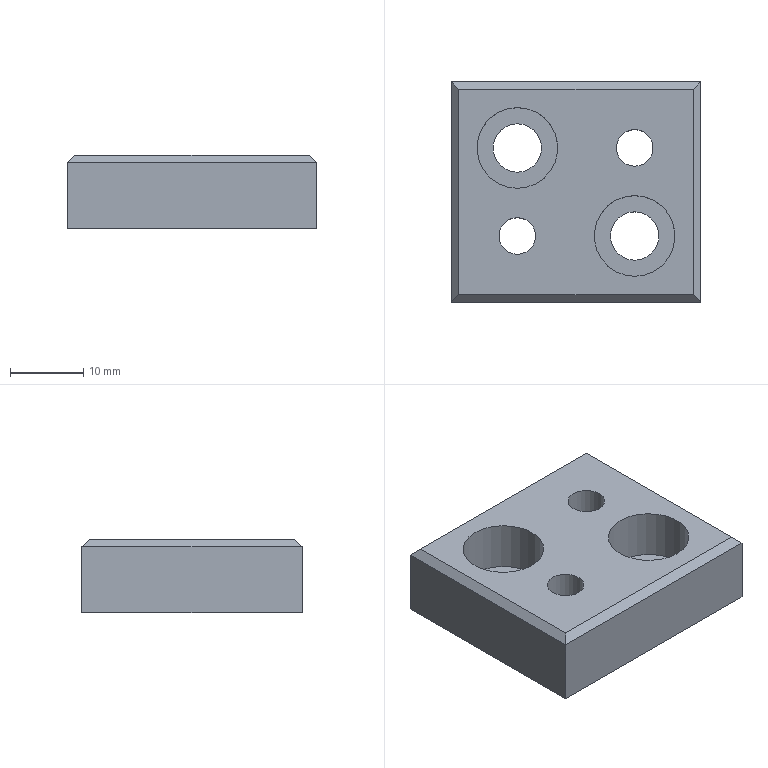Component | NX | SQUARE_TOOL_BLOCK | 1 solid | 18 faces | volume 8233 mm3 | plane 12 | cylinder 6 | commonest cylinder face diameters 6.6 x2 11 x2 5 x2